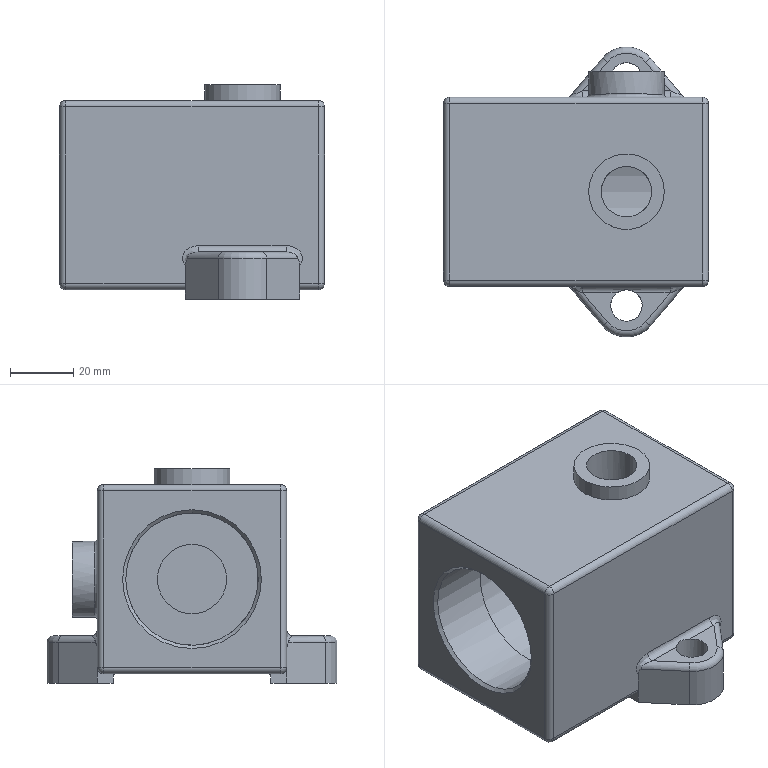Component | NX | PUMP_BODY | 1 solid | 74 faces | volume 202911 mm3 | cylinder 33 | plane 25 | sphere 8 | spline 4 | torus 3 | cone 1 | commonest cylinder face diameters 4 x20 20 x2 2 x2 24 x2 16 x2 10 x2 45 x1 42 x1